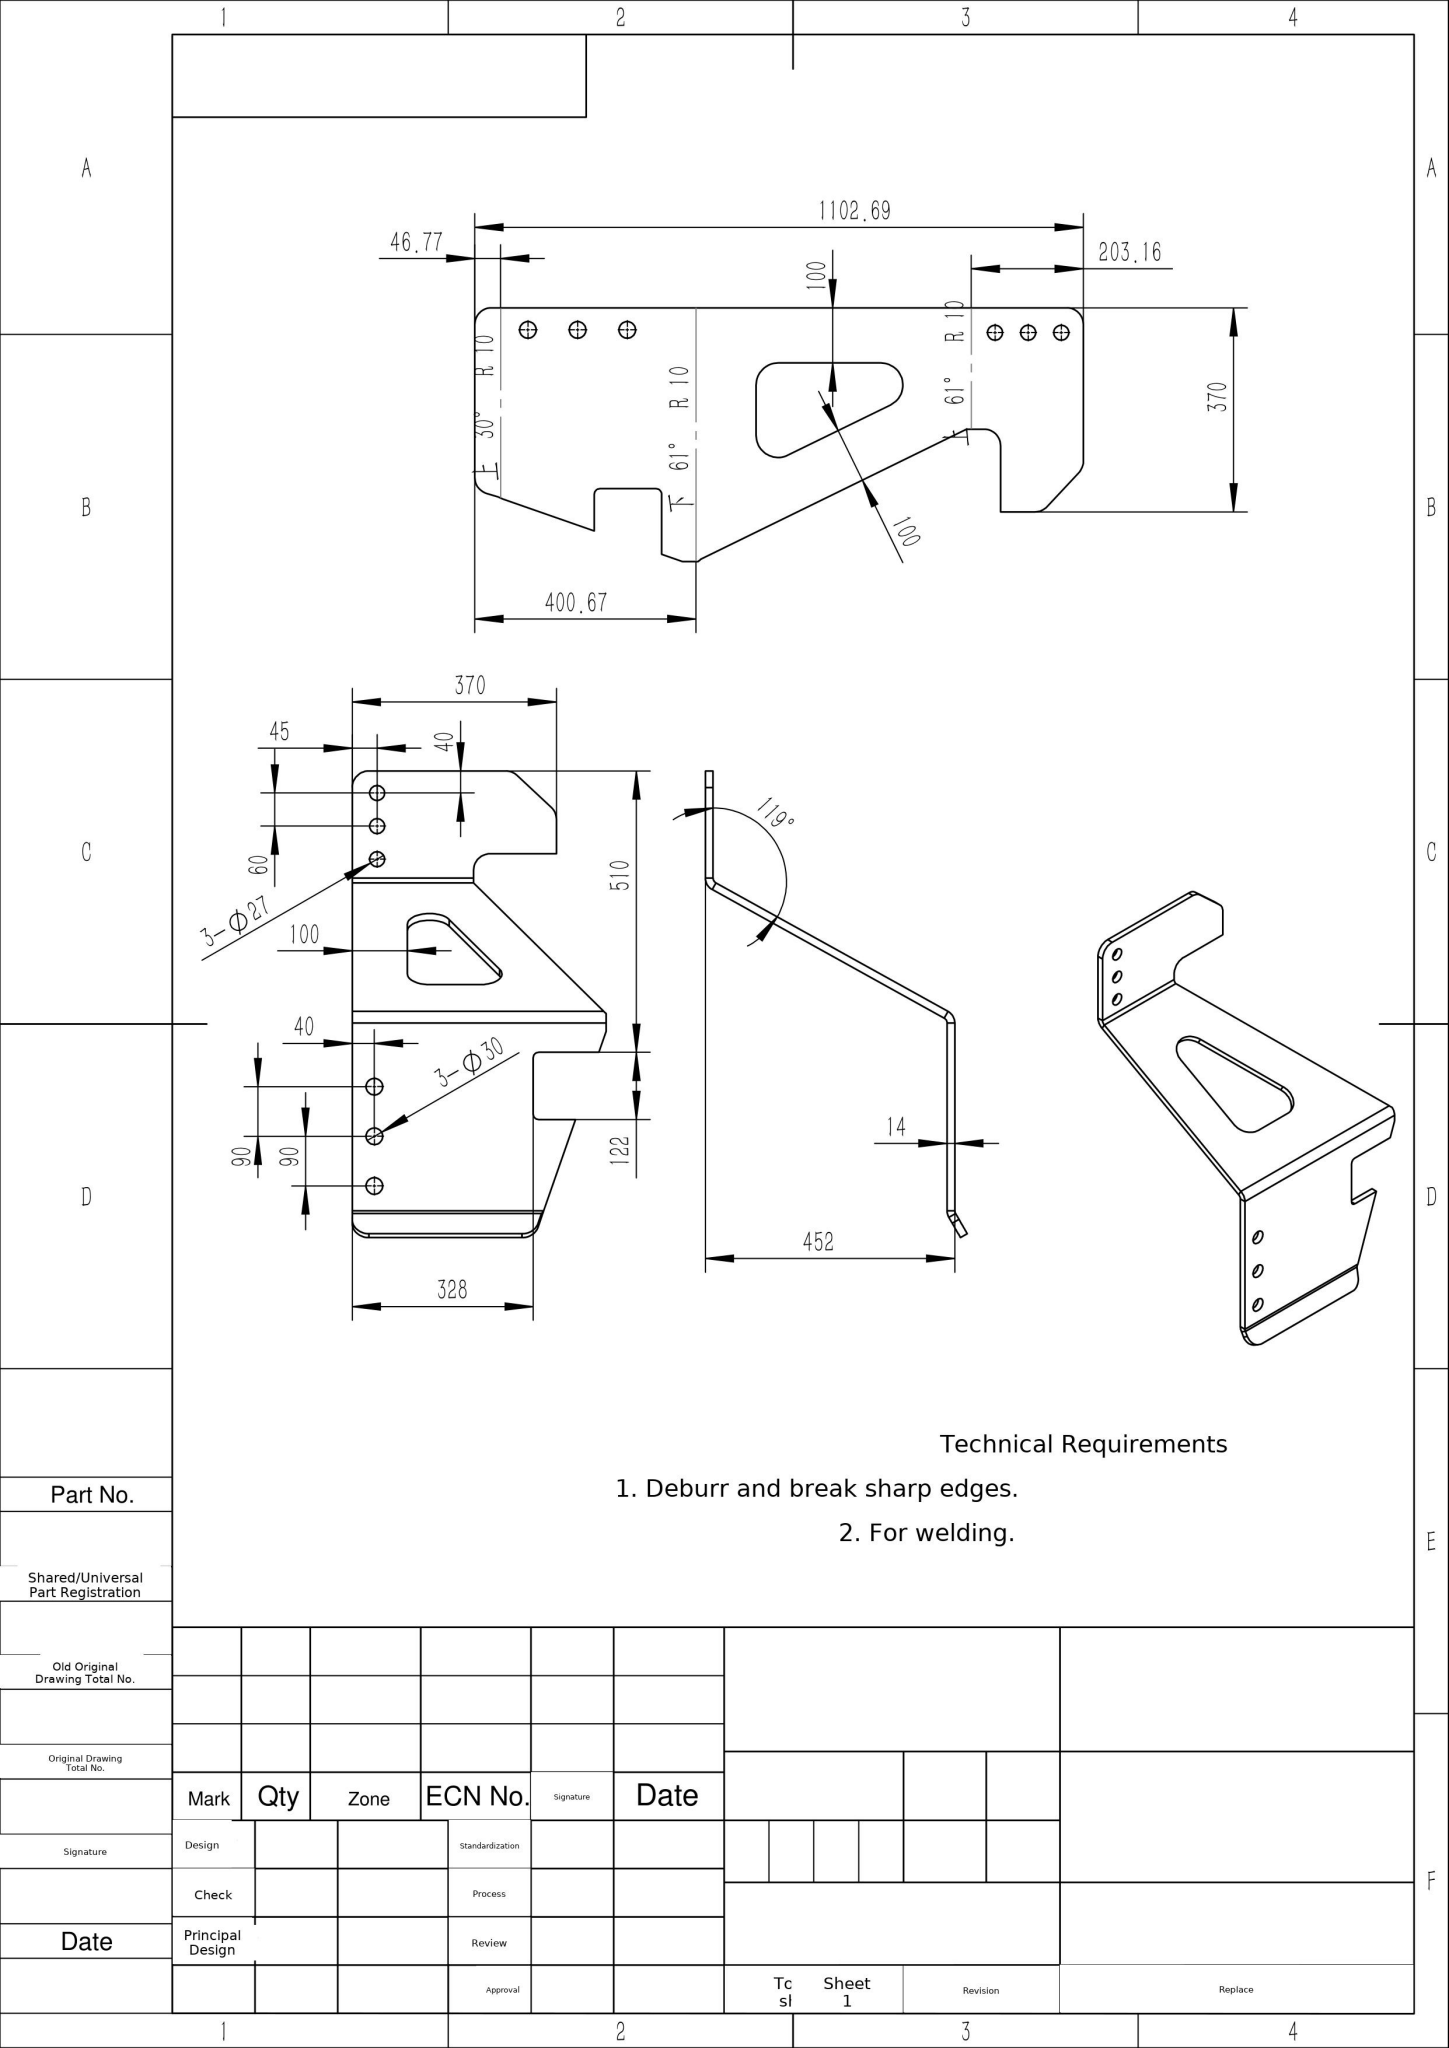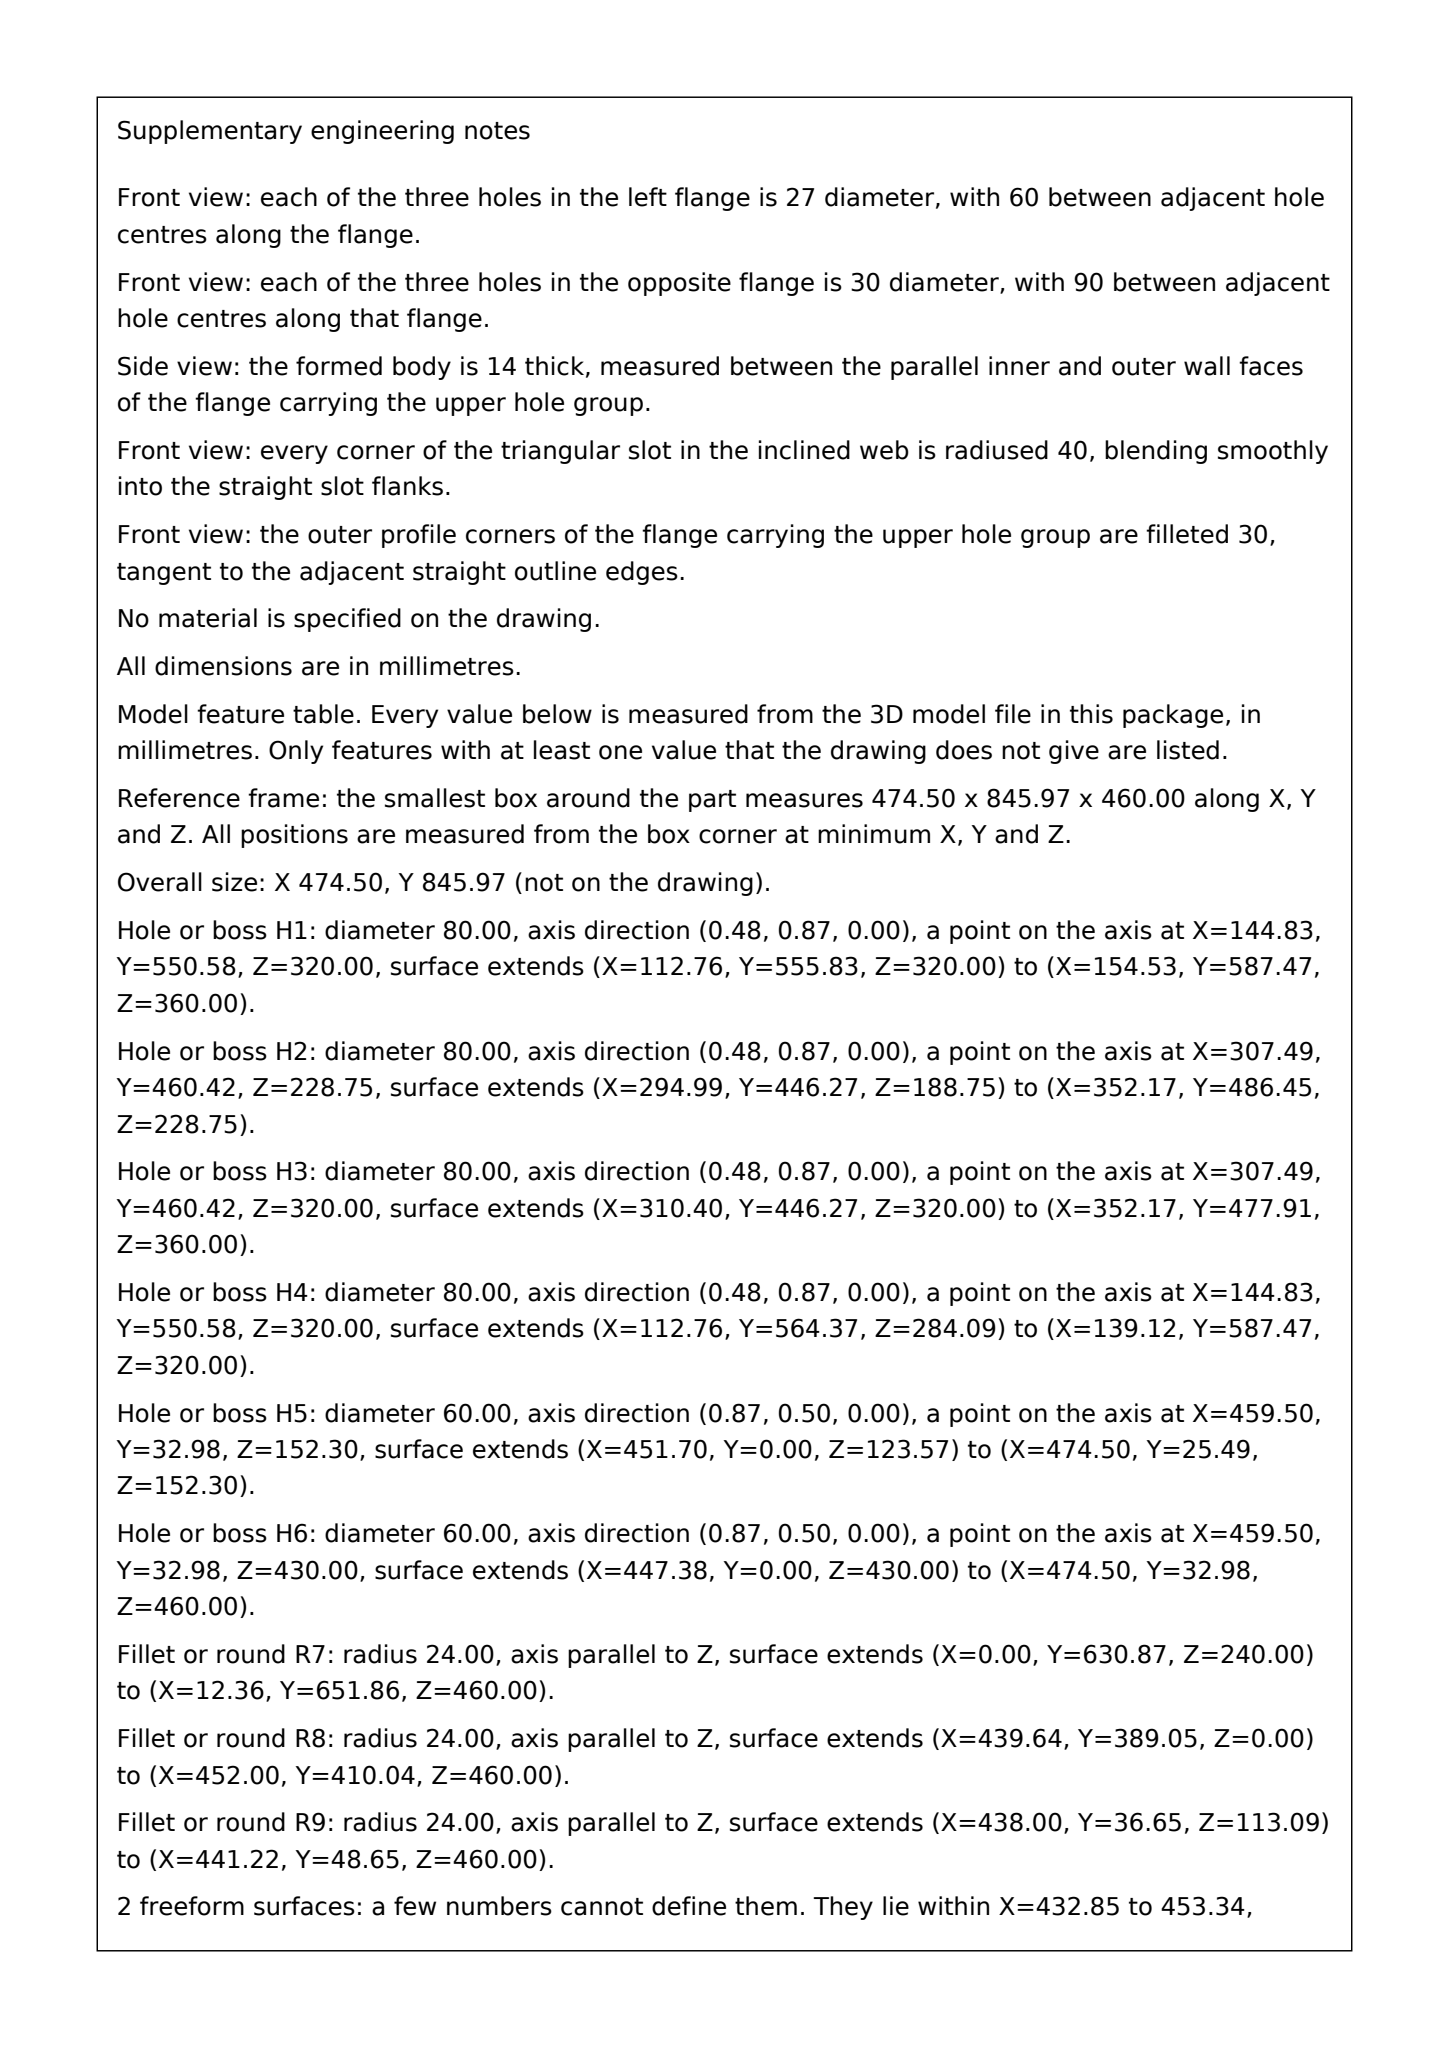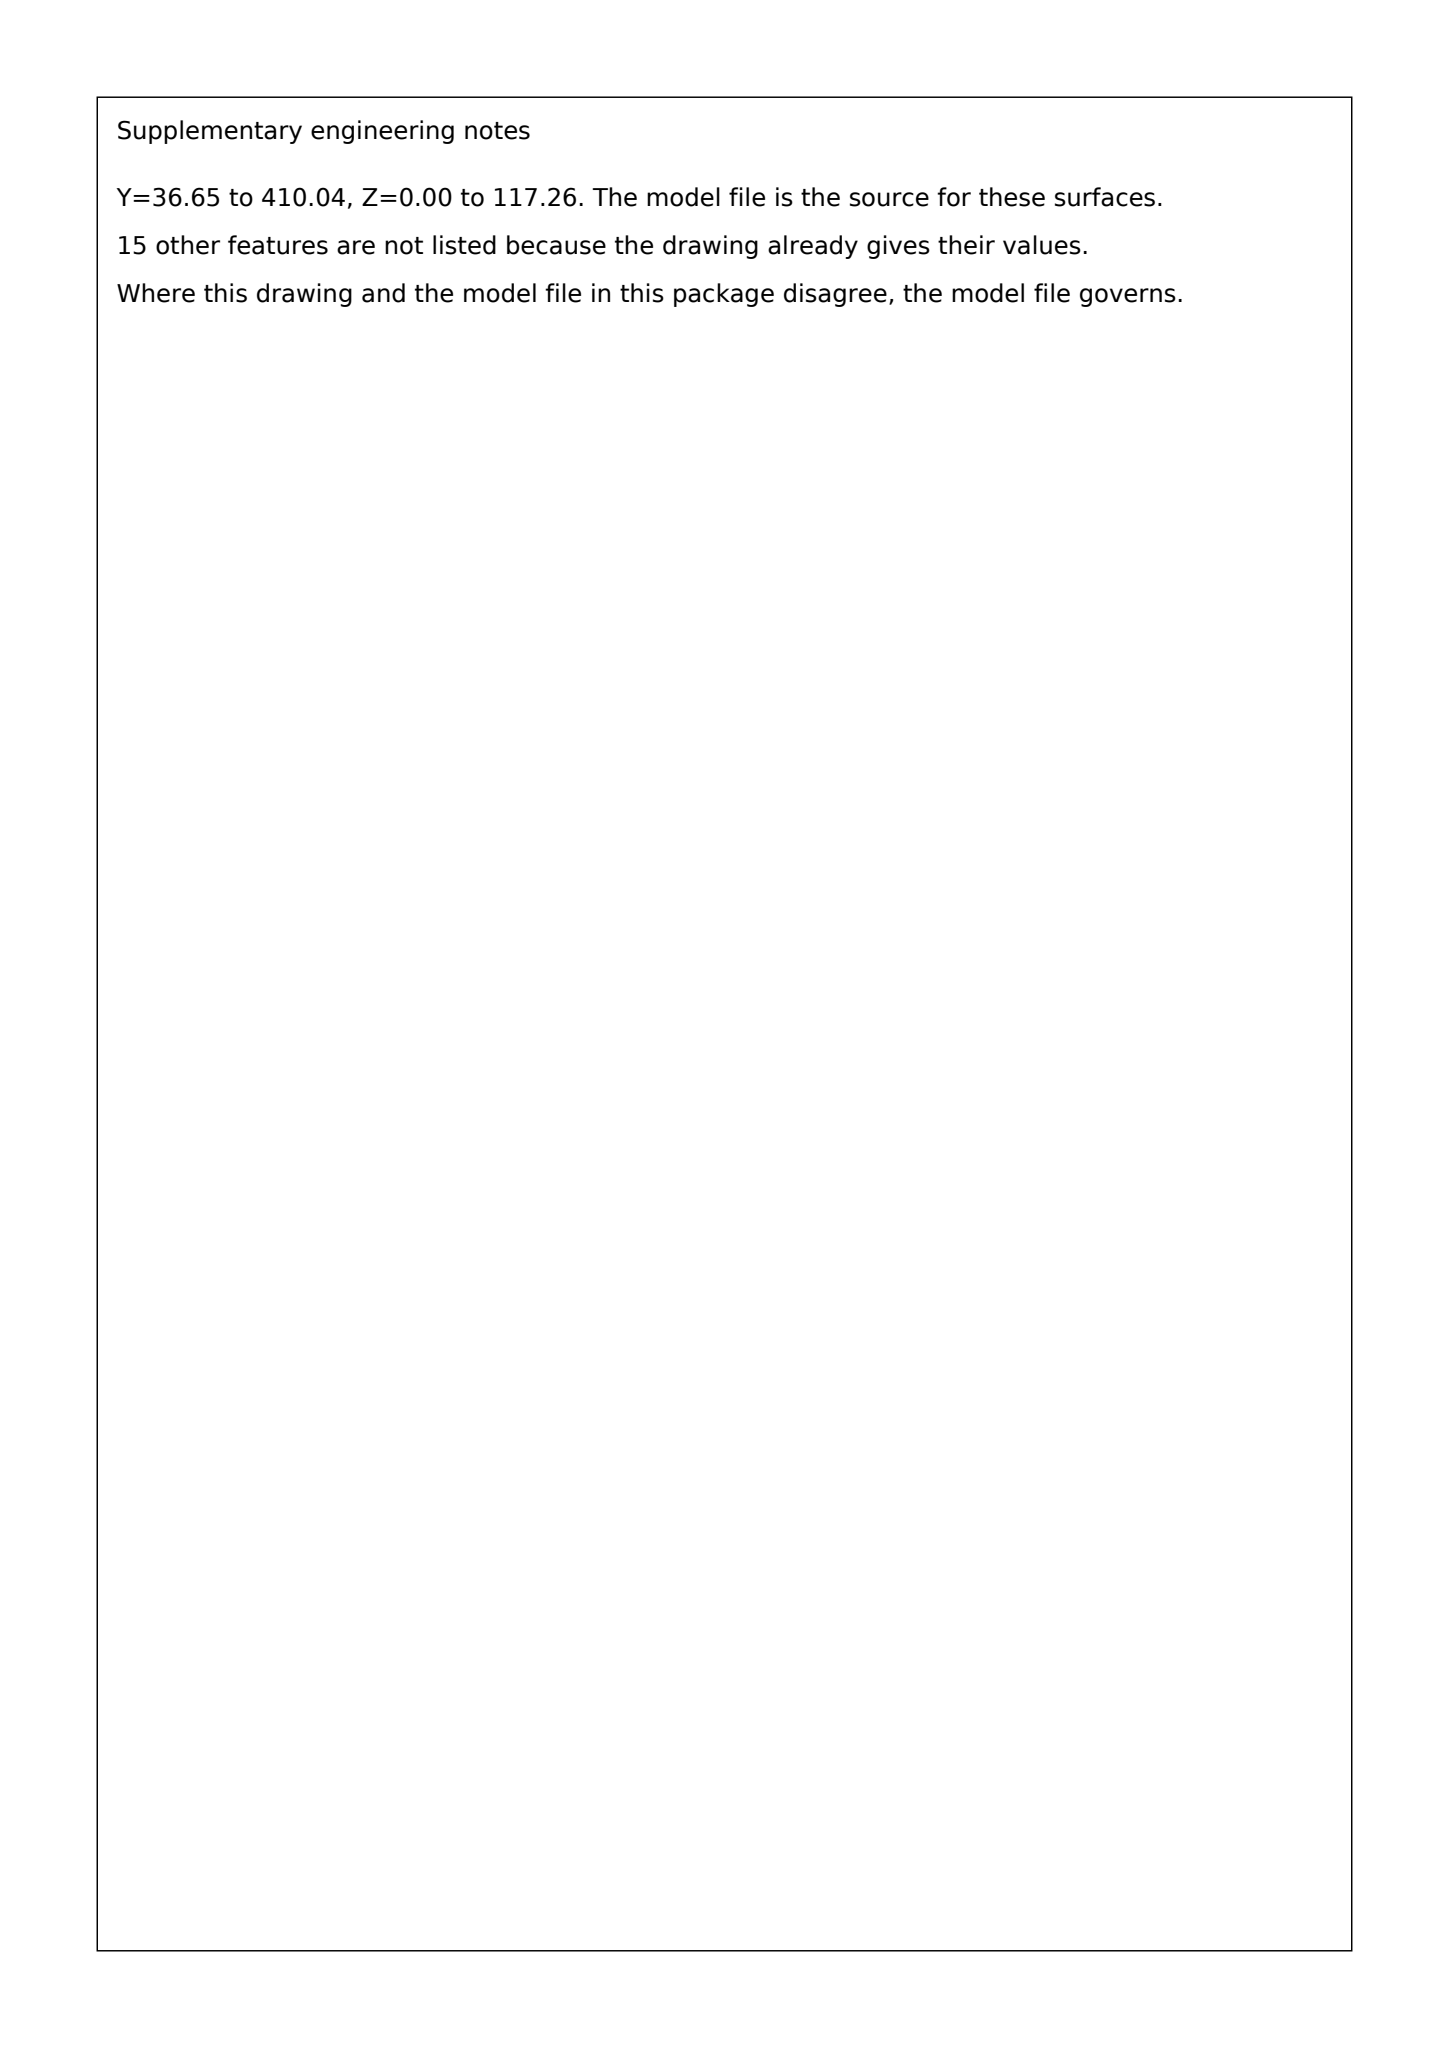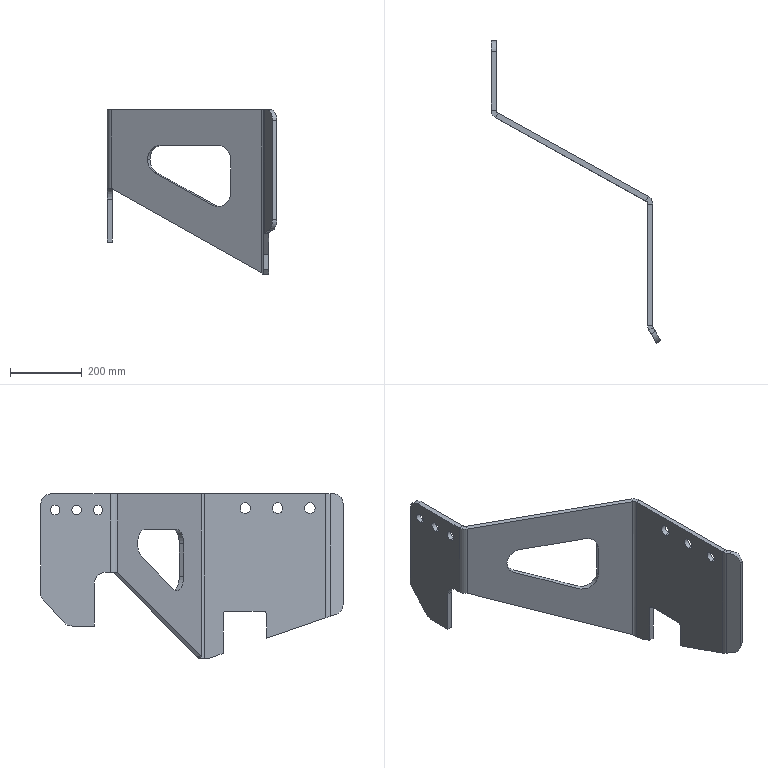Part | SolidWorks | mm | 1 solid | 66 faces | box 474.5 x 845.97 x 460 mm | volume 4809898 mm3 | plane 34 | cylinder 30 | spline 2 | commonest cylinder face diameters 27 x6 30 x6 60 x6 20 x5 80 x4 48 x3
Drawing notes:
SLOT: 3X R40 BLENDED, CTR SPACING 162.66 x 91.25, 242.66 OAL | from the solid: Ø80 y-axis cyls at (x,z)=(144.83,361.42),(307.49,361.42),(307.49,270.17): 3X R40, ctr dist 162.66 and 91.25; overall 162.66+80=242.66 x 91.25+80=171.25
SLOT OVERALL 242.66 x 171.25, LEGS PARALLEL TO VIEW AXES | from the solid: Slot arc centres share x=307.49 and z=361.42, so leg lines are axis-parallel; sizes from R40 centres + 2x40
NOTCH 122 WIDE x 42 DP, R10 CNRS, 213.97 FROM BOTTOM EDGE | from the solid: y-planes 213.97 & 335.97 (=122 wide); z-planes 173.42 (notch floor) vs 131.42 (edge) =42 dp; Ø20 x-axis cyls at (223.97,163.42) & (325.97,163.42) = R10 inner corners; lower edge y=0
UNSPECIFIED OUTLINE CORNER RADII R30 | from the solid: 6X Ø60 x-axis cyls on profile corners: (32.98,193.72),(32.98,471.42),(665.97,251.42),(758.33,161.42),(815.97,223.23),(815.97,471.42)
3-Ø27 EQ SP 60 (2 X 60 = 120) | from the solid: Ø27 holes at y=685.97, 745.97, 805.97, z=456.42 -> equal 60 pitch
3-Ø27 GROUP: TOP HOLE 40 FROM TOP EDGE, 45 FROM LH EDGE | from the solid: Top Ø27 y=805.97 vs top edge y=845.97 =40; z=456.42 vs edge z=501.42 =45
3-Ø30 GROUP: LOWEST HOLE 93.65 FROM BOTTOM EDGE | from the solid: Ø30 holes y=93.65/183.65/273.65 (90 pitch), bbox min y=0; z=461.42 vs edge 501.42 =40
OVERALL DEPTH 476; END FLANGE 14 THK, FACES 438 & 452 | from the solid: bbox x=476.0; x-planes 0, 14, 438, 452 (14 thk plates at each end)
UPPER FLANGE STEP 122 HIGH, TOP 335.97 FROM BOTTOM EDGE | from the solid: y-planes 335.97 and 213.97 (step 122), bottom datum y=0; 845.97-335.97=510 agrees with existing 510 dim
MAX PROFILE DEPTH 501.4 FROM BACK DATUM EDGE (370/328 ORIGIN) | from the solid: bbox Z = 501.417; back datum face Z=501.42 (7 faces), deepest profile point at Z=0; existing 370 -> Z=131.42, 328 -> Z=173.42